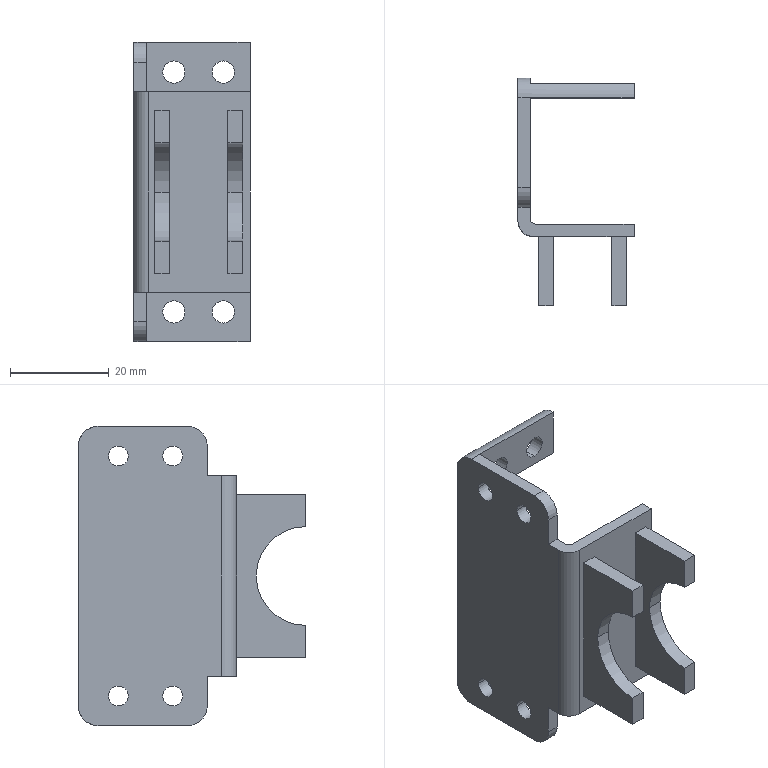Component | SolidWorks | Bracket-1 | 1 solid | 60 faces | volume 9254 mm3 | plane 34 | cylinder 26 | commonest cylinder face diameters 4.5 x8 4 x8 20 x4 8 x4 6 x1 2 x1 | material 45